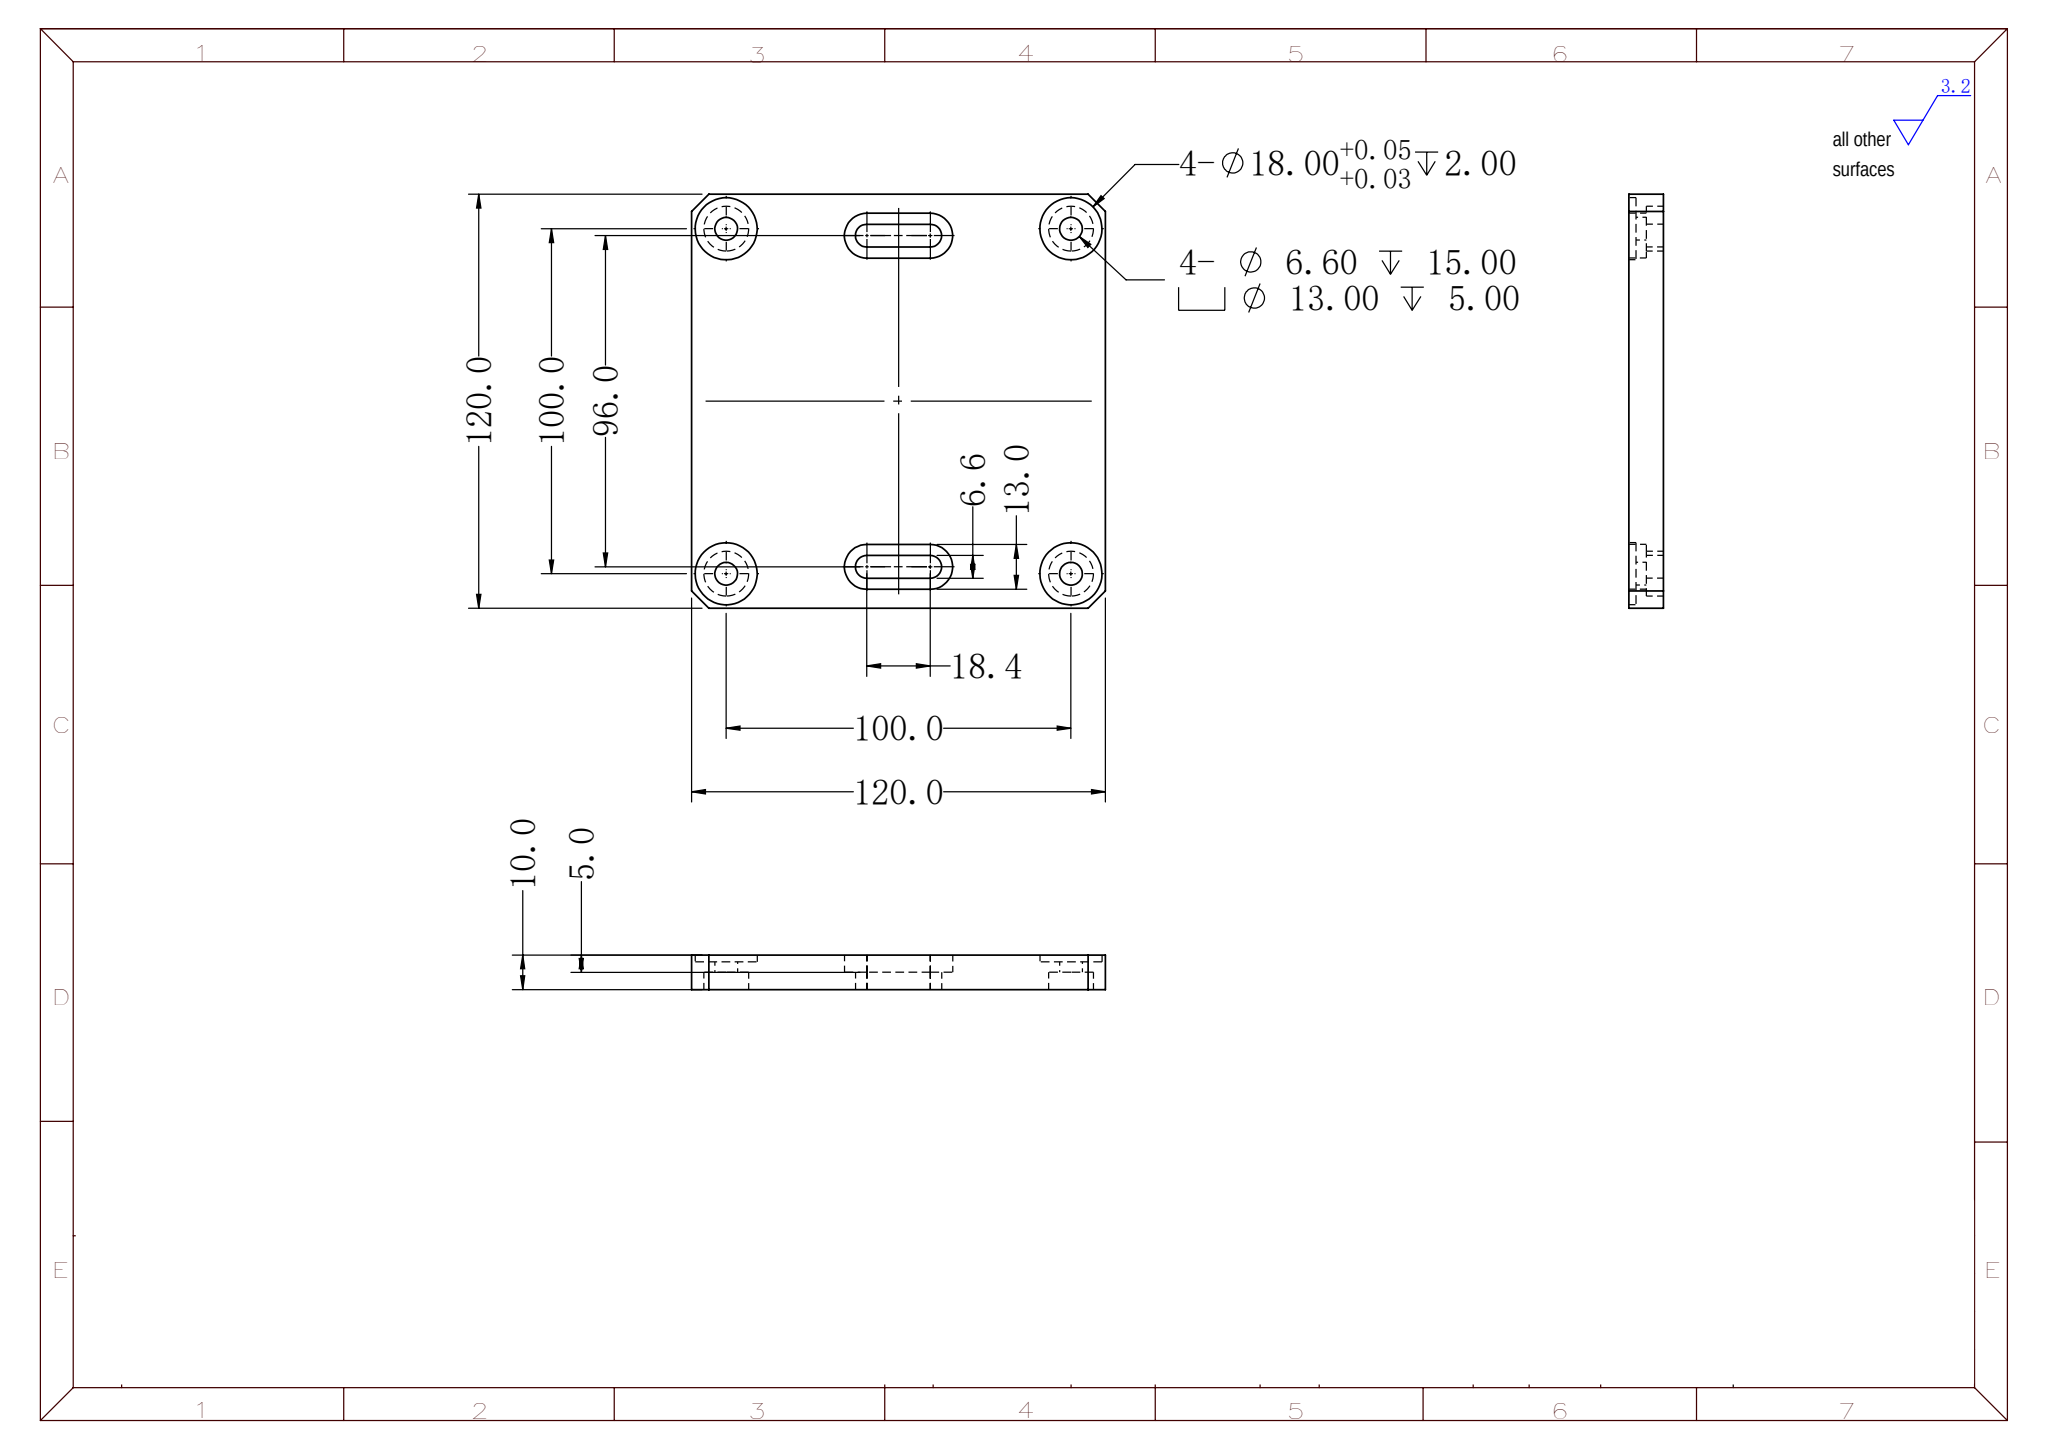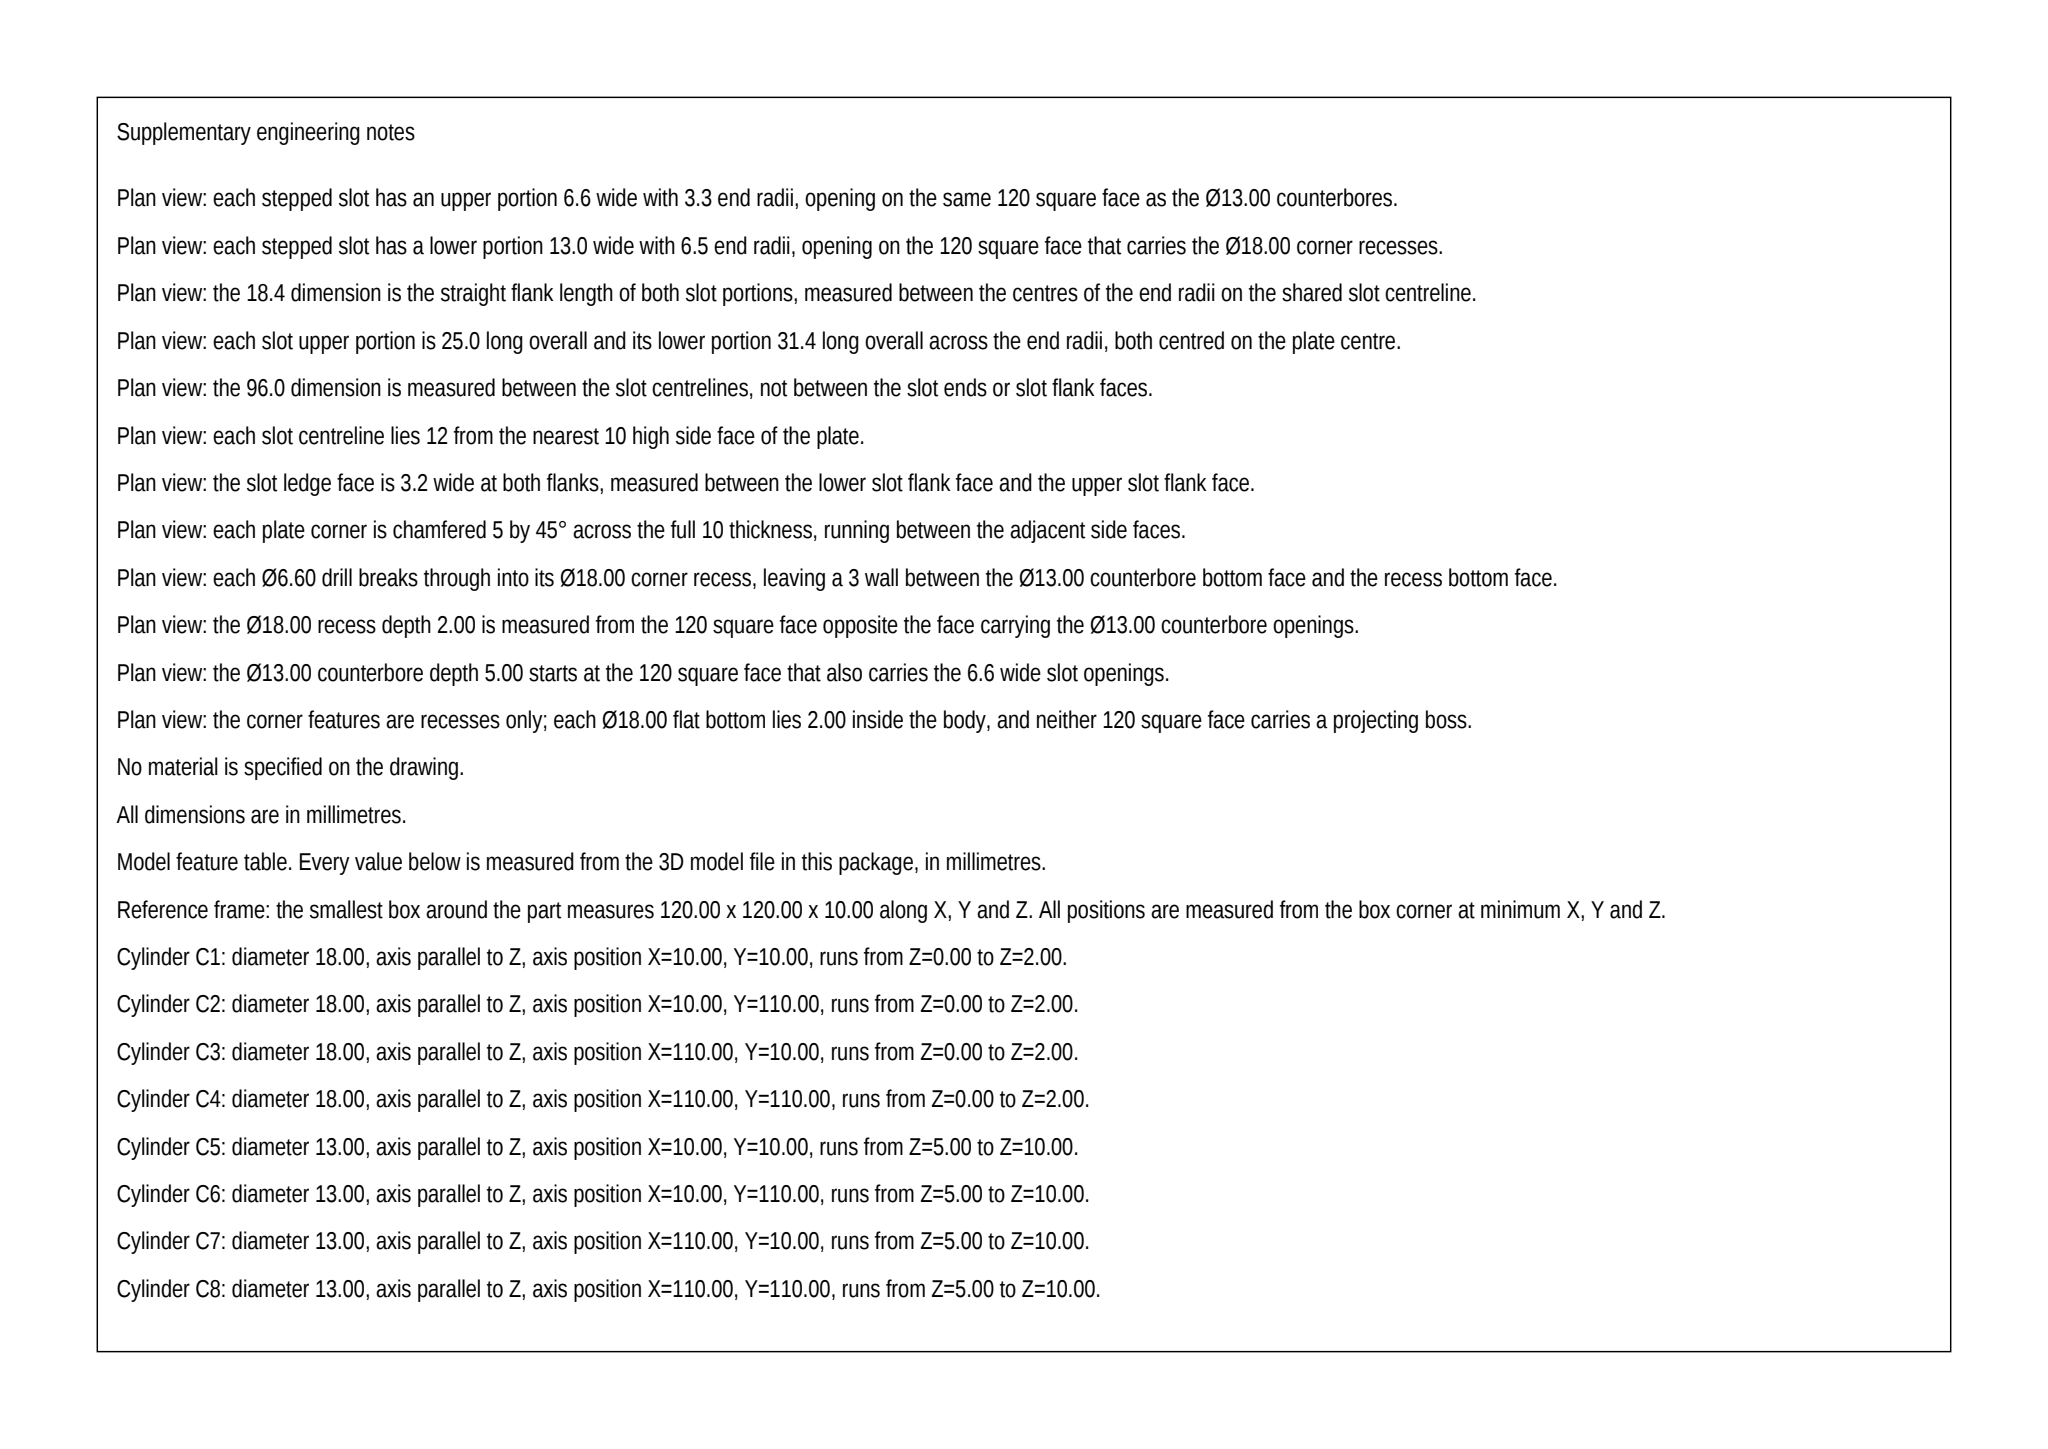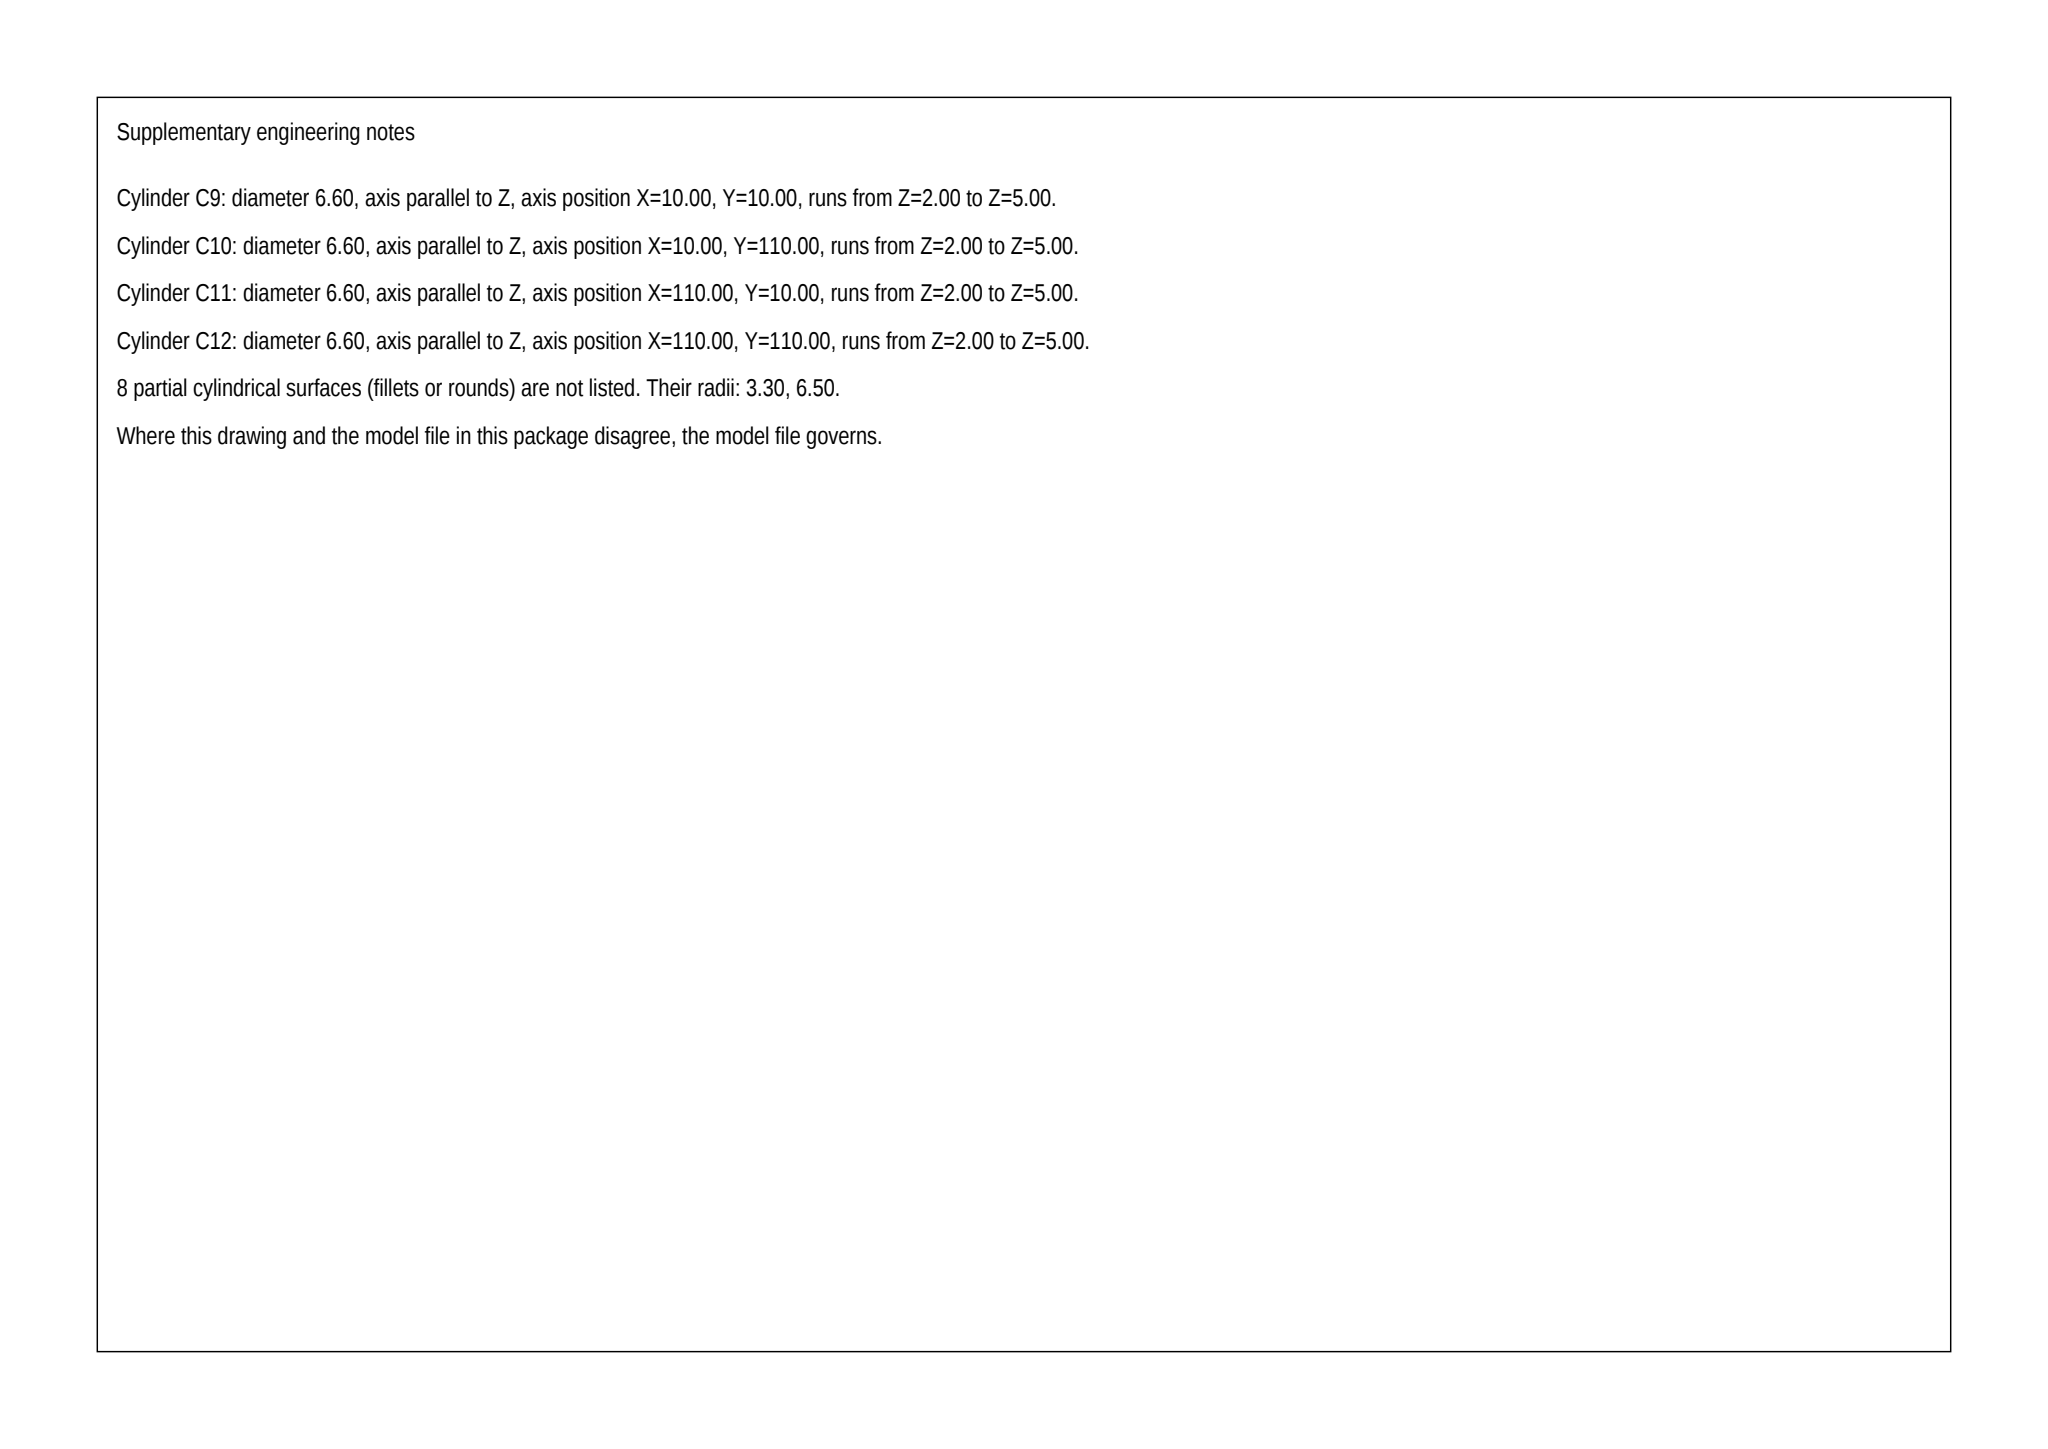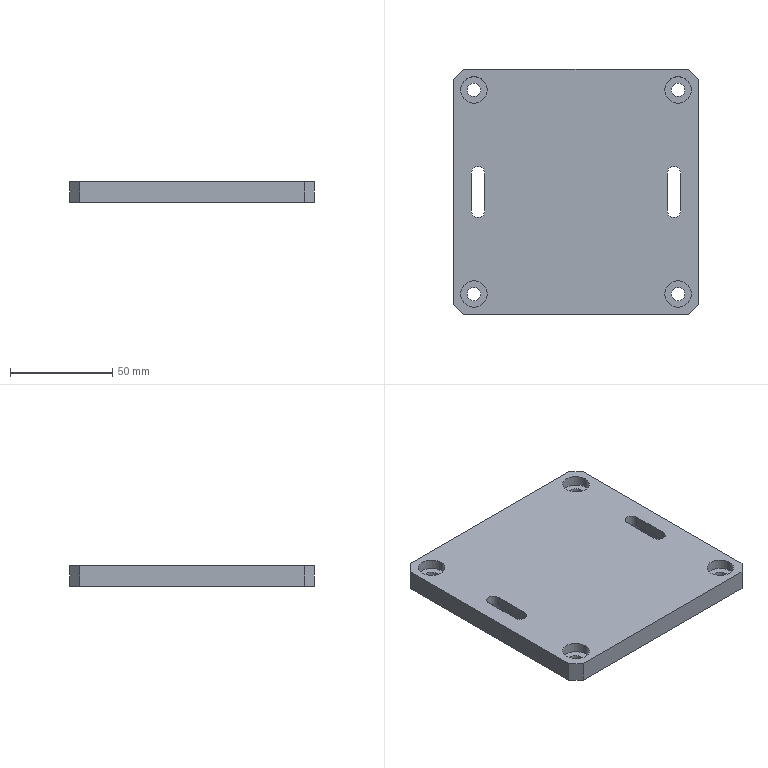Part | SolidWorks | mm | 1 solid | 60 faces | box 120 x 120 x 10 mm | volume 133123 mm3 | cylinder 32 | plane 28 | commonest cylinder face diameters 13 x12 6.6 x12 18 x8
Drawing notes:
4X Ø18.00 DP 2.00 + CBORE Ø13.00 DP 5.00 ALSO ON OPP FACE, 8 PLCS EA | from the solid: Ø18 L=2 count 2 and Ø13 L=5 count 2 at each corner axis (10,10),(10,110),(110,10),(110,110); z-planes at 2.0 (4) and 5.0 (6) from both faces
2X SLOT: Ø6.60 THRU, 18.4 C-C; CBORE Ø13.00 DP 5.00 | from the solid: Ø6.6 cyl L=5.0 at (12,50.8)/(12,69.2)/(108,50.8)/(108,69.2) + Ø13 cyl L=5.0 same axes; 5+5=10 = plate thk, so 6.6 is thru; c-c 69.2-50.8=18.4
SLOT CBORE Ø13.00 DP 5.00 ONE FACE ONLY - NOT OPP FACE | from the solid: Only one Ø13 c'bore per slot end (count 1 each) vs count 2 at corner holes; c'bore floor at z=5.0 (z-plane offset 5.0, 6 instances) of 10.0 thk plate
SLOT CBORE ON SAME FACE AS 4X Ø13.00 CORNER CBORE | from the solid: Slot Ø13 floors and corner Ø13 floors share z=5.0 plane; Ø18 ↧2.0 bores on opposite face (z-plane 2.0, 4 instances)
4X C5 AT PLATE CORNERS - IGNORE STRAY '11' | from the solid: 120x120x10 bbox, fillet_radii empty (flat corner cuts, not radii); corner break per drawing C5